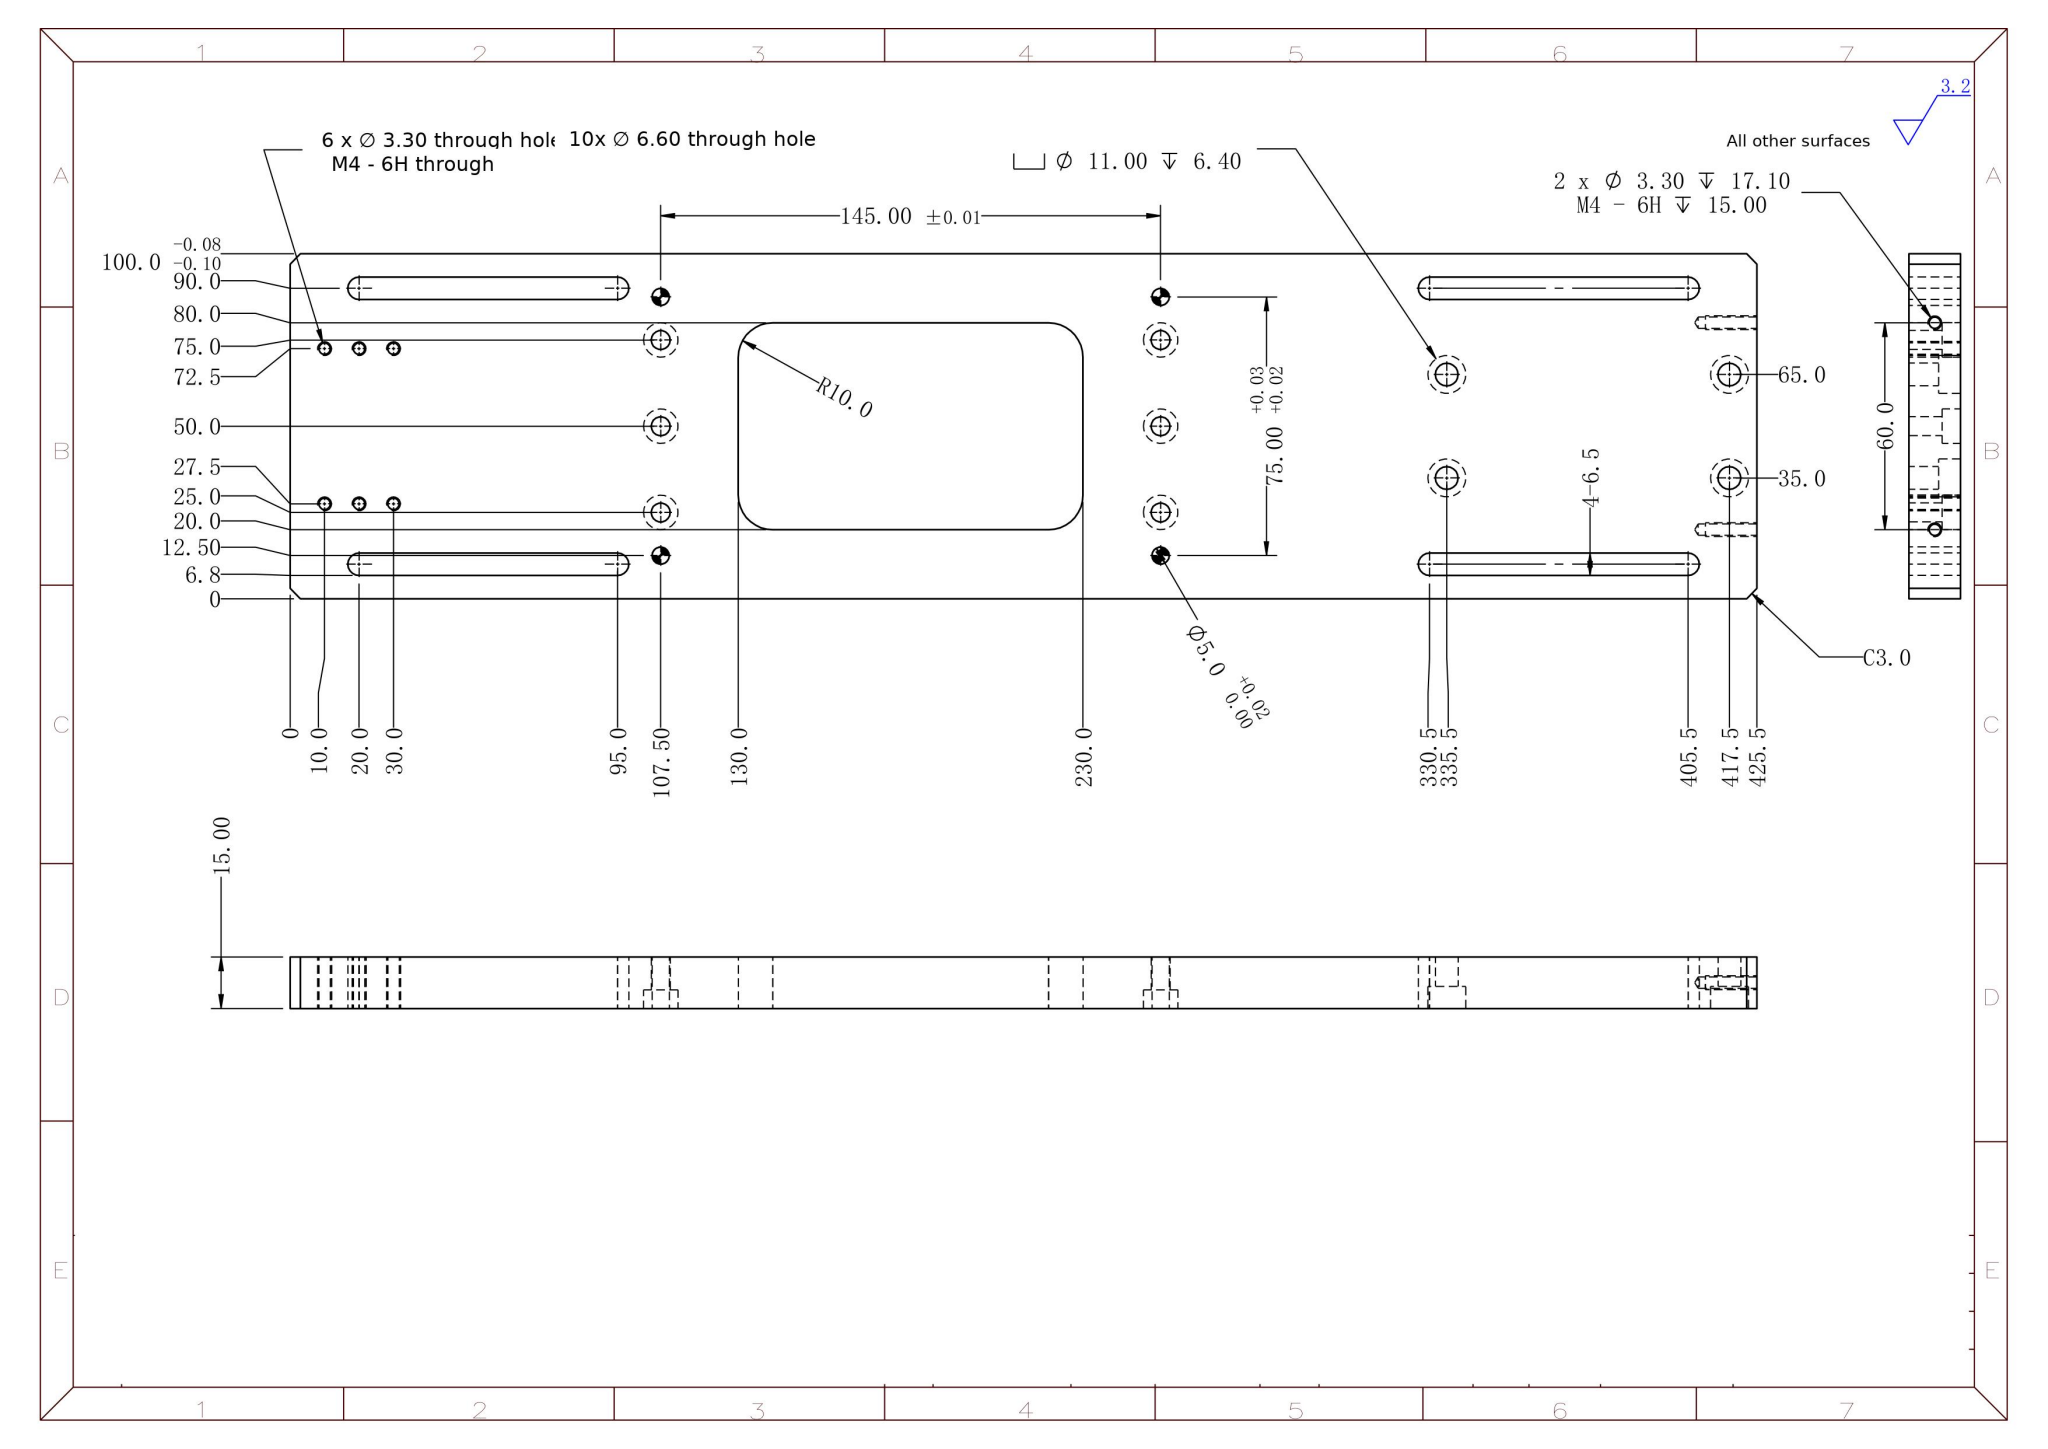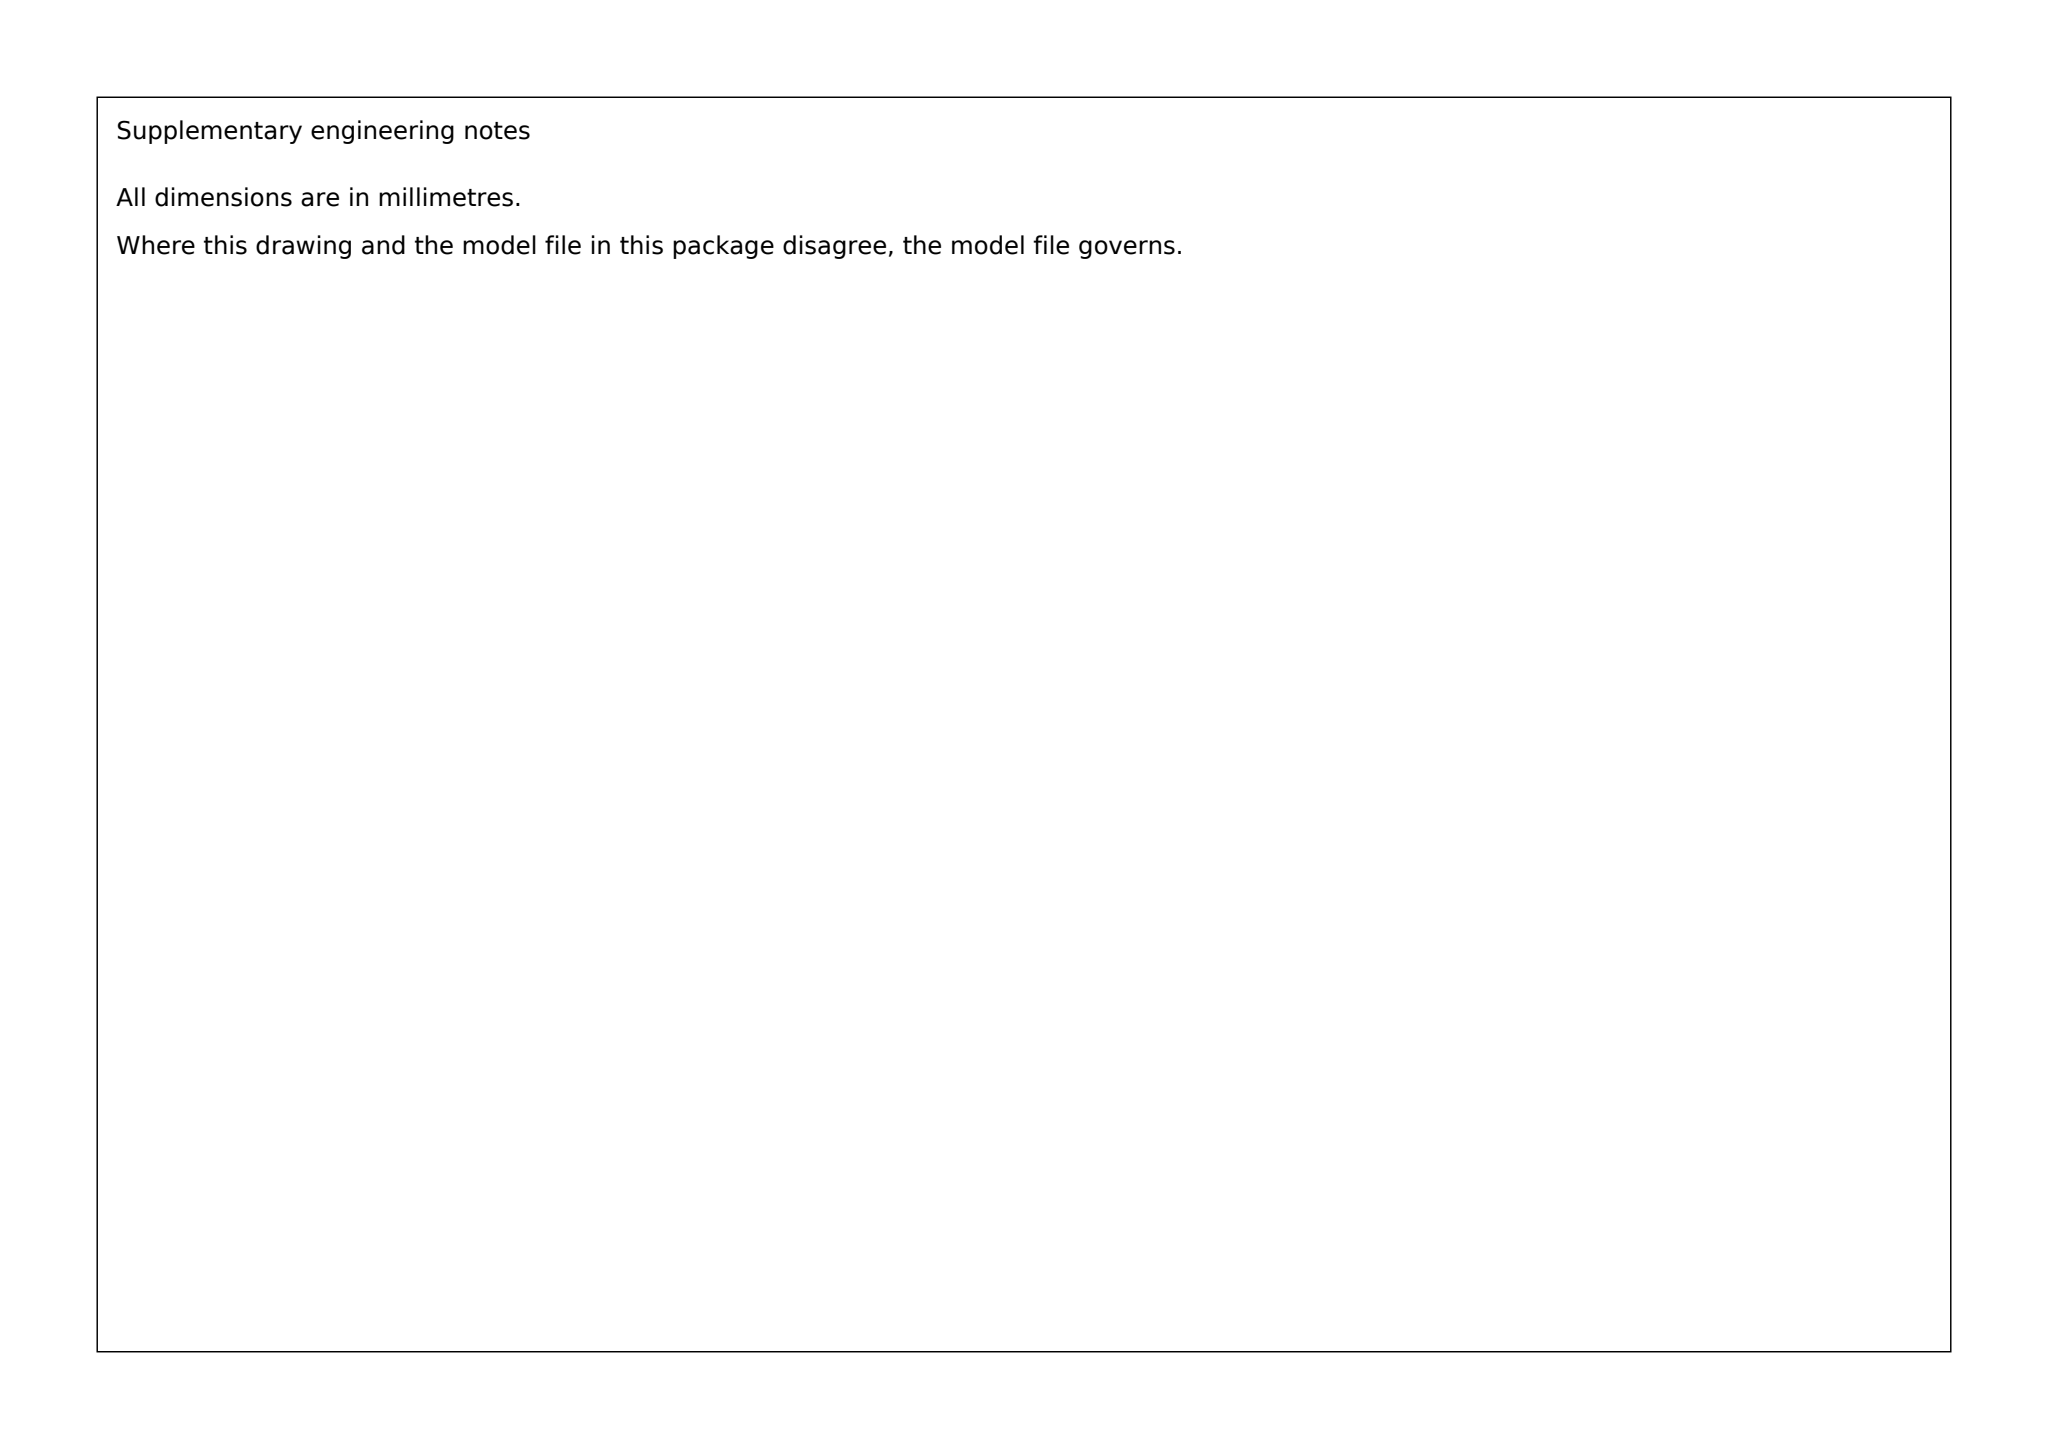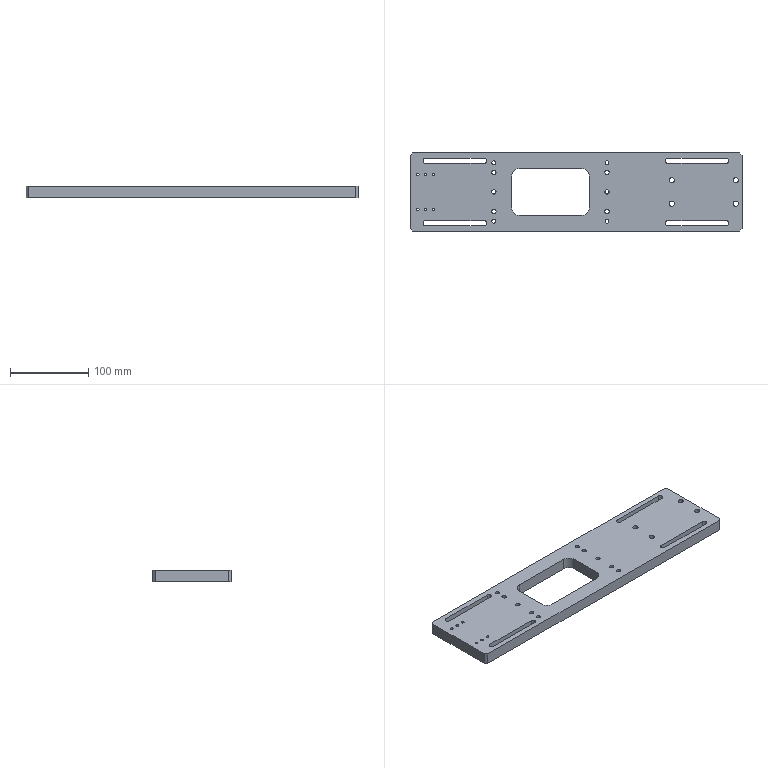Part | SolidWorks | mm | 1 solid | 116 faces | box 425.5 x 100 x 15 mm | volume 508258 mm3 | cylinder 80 | plane 32 | cone 4 | commonest cylinder face diameters 3.3 x16 6.5 x12 10 x12 5.5 x12 5 x8 11 x8 6.6 x8 20 x4
build123d program:
from build123d import *

# Parameters (mm, degrees)
SKETCH1_W                                       = 425.5
SKETCH1_H                                       = 100
BOSS_EXTRUDE1_DEPTH                             = 7.5
CHAMFER1_SIZE                                   = 3
M6_HEX_SOCKET_HEAD_CAP_SCREW_CBORE1_D           = 6.6
M6_HEX_SOCKET_HEAD_CAP_SCREW_CBORE1_CBORE_D     = 11
M6_HEX_SOCKET_HEAD_CAP_SCREW_CBORE1_CBORE_DEPTH = 6.4
SKETCH10_R                                      = 2.5
CUT_EXTRUDE3_DEPTH                              = 220.061
SKETCH11_W                                      = 100
SKETCH11_H                                      = 60
CUT_EXTRUDE4_DEPTH                              = 220.061
FILLET1_R                                       = 10
M5_HEX_SOCKET_HEAD_CAP_SCREW_CBORE2_D           = 5.5
M5_HEX_SOCKET_HEAD_CAP_SCREW_CBORE2_DEPTH       = 16.6
M5_HEX_SOCKET_HEAD_CAP_SCREW_CBORE2_CBORE_D     = 10
M5_HEX_SOCKET_HEAD_CAP_SCREW_CBORE2_CBORE_DEPTH = 5.4
M5_HEX_SOCKET_HEAD_CAP_SCREW_CBORE2_TIP         = 1.652
M4_TAPPED_HOLE1_D                               = 3.3
CUT_EXTRUDE5_DEPTH                              = 220.061
M4_TAPPED_HOLE2_D                               = 3.3
M4_TAPPED_HOLE2_DEPTH                           = 17.1
M4_TAPPED_HOLE2_TIP                             = 0.9914


with BuildPart() as part:
    # Sketch1 → Boss-Extrude1 (new, symmetric)
    with BuildSketch(Plane.XY):
        Rectangle(SKETCH1_W, SKETCH1_H)
    extrude(amount=BOSS_EXTRUDE1_DEPTH, both=True)

    # Chamfer1
    chamfer1_edges = [part.edges().sort_by_distance(p)[0] for p in [
        (212.75, -50, 0),
        (-212.75, -50, 0),
        (-212.75, 50, 0),
        (212.75, 50, 0),
    ]]
    chamfer(chamfer1_edges, length=CHAMFER1_SIZE)

    # M6 Hex Socket Head Cap Screw CBORE1 (through all)
    with Locations(Plane(origin=(0, 0, -7.5), x_dir=(-1, 0, 0), z_dir=(0, 0, -1))):
        with Locations((-204.75, 15), (-122.75, 15), (-122.75, -15), (-204.75, -15)):
            CounterBoreHole(M6_HEX_SOCKET_HEAD_CAP_SCREW_CBORE1_D / 2, M6_HEX_SOCKET_HEAD_CAP_SCREW_CBORE1_CBORE_D / 2, M6_HEX_SOCKET_HEAD_CAP_SCREW_CBORE1_CBORE_DEPTH)

    # Sketch10 → Cut-Extrude3 (cut, through all)
    with BuildSketch(Plane.XY.offset(7.5)):
        with Locations((-105.25, 37.5)):
            Circle(SKETCH10_R)
        with Locations((39.75, 37.5)):
            Circle(SKETCH10_R)
        with Locations((39.75, -37.5)):
            Circle(SKETCH10_R)
        with Locations((-105.25, -37.5)):
            Circle(SKETCH10_R)
    extrude(amount=-CUT_EXTRUDE3_DEPTH, mode=Mode.SUBTRACT)

    # Sketch11 → Cut-Extrude4 (cut, through all)
    with BuildSketch(Plane.XY.offset(7.5)):
        with Locations((-32.75, 0)):
            Rectangle(SKETCH11_W, SKETCH11_H)
    extrude(amount=-CUT_EXTRUDE4_DEPTH, mode=Mode.SUBTRACT)

    # Fillet1
    fillet1_edges = [part.edges().sort_by_distance(p)[0] for p in [
        (17.25, 30, 0),
        (17.25, -30, 0),
        (-82.75, -30, 0),
        (-82.75, 30, 0),
    ]]
    fillet(fillet1_edges, radius=FILLET1_R)

    # M5 Hex Socket Head Cap Screw CBORE2
    with Locations(Plane(origin=(0, 0, -7.5), x_dir=(-1, 0, 0), z_dir=(0, 0, -1))):
        with Locations((-39.75, 25), (-39.75, 0), (-39.75, -25), (105.25, 25), (105.25, 0), (105.25, -25)):
            CounterBoreHole(M5_HEX_SOCKET_HEAD_CAP_SCREW_CBORE2_D / 2, M5_HEX_SOCKET_HEAD_CAP_SCREW_CBORE2_CBORE_D / 2, M5_HEX_SOCKET_HEAD_CAP_SCREW_CBORE2_CBORE_DEPTH, depth=M5_HEX_SOCKET_HEAD_CAP_SCREW_CBORE2_DEPTH)
            with Locations((0, 0, -(M5_HEX_SOCKET_HEAD_CAP_SCREW_CBORE2_DEPTH + M5_HEX_SOCKET_HEAD_CAP_SCREW_CBORE2_TIP / 2))):  # 118° drill point
                Cone(0, M5_HEX_SOCKET_HEAD_CAP_SCREW_CBORE2_D / 2, M5_HEX_SOCKET_HEAD_CAP_SCREW_CBORE2_TIP, mode=Mode.SUBTRACT)

    # M4 Tapped Hole1 (through all)
    with Locations(Plane.XY.offset(7.5)):
        with Locations((-192.75, -22.5), (-202.75, -22.5), (-182.75, -22.5), (-182.75, 22.5), (-192.75, 22.5), (-202.75, 22.5)):
            Hole(M4_TAPPED_HOLE1_D / 2)

    # Sketch18 → Cut-Extrude5 (cut, through all)
    with BuildSketch(Plane.XY.offset(7.5)):
        with BuildLine():
            Line((192.75, -43.25), (117.75, -43.25))
            ThreePointArc((117.75, -43.25), (114.5, -40), (117.75, -36.75))
            Line((117.75, -36.75), (192.75, -36.75))
            ThreePointArc((192.75, -36.75), (196, -40), (192.75, -43.25))
        make_face()
        with BuildLine():
            Line((192.75, 43.25), (117.75, 43.25))
            ThreePointArc((117.75, 43.25), (114.5, 40), (117.75, 36.75))
            Line((117.75, 36.75), (192.75, 36.75))
            ThreePointArc((192.75, 36.75), (196, 40), (192.75, 43.25))
        make_face()
        with BuildLine():
            Line((-192.75, -43.25), (-117.75, -43.25))
            ThreePointArc((-117.75, -43.25), (-114.5, -40), (-117.75, -36.75))
            Line((-117.75, -36.75), (-192.75, -36.75))
            ThreePointArc((-192.75, -36.75), (-196, -40), (-192.75, -43.25))
        make_face()
        with BuildLine():
            Line((-192.75, 43.25), (-117.75, 43.25))
            ThreePointArc((-117.75, 43.25), (-114.5, 40), (-117.75, 36.75))
            Line((-117.75, 36.75), (-192.75, 36.75))
            ThreePointArc((-192.75, 36.75), (-196, 40), (-192.75, 43.25))
        make_face()
    extrude(amount=-CUT_EXTRUDE5_DEPTH, mode=Mode.SUBTRACT)

    # M4 Tapped Hole2
    with Locations(Plane(origin=(212.75, 0, 0), x_dir=(0, 0, -1), z_dir=(1, 0, 0))):
        with Locations((0, 30), (0, -30)):
            Hole(M4_TAPPED_HOLE2_D / 2, depth=M4_TAPPED_HOLE2_DEPTH)
            with Locations((0, 0, -(M4_TAPPED_HOLE2_DEPTH + M4_TAPPED_HOLE2_TIP / 2))):  # 118° drill point
                Cone(0, M4_TAPPED_HOLE2_D / 2, M4_TAPPED_HOLE2_TIP, mode=Mode.SUBTRACT)


solid = part.part